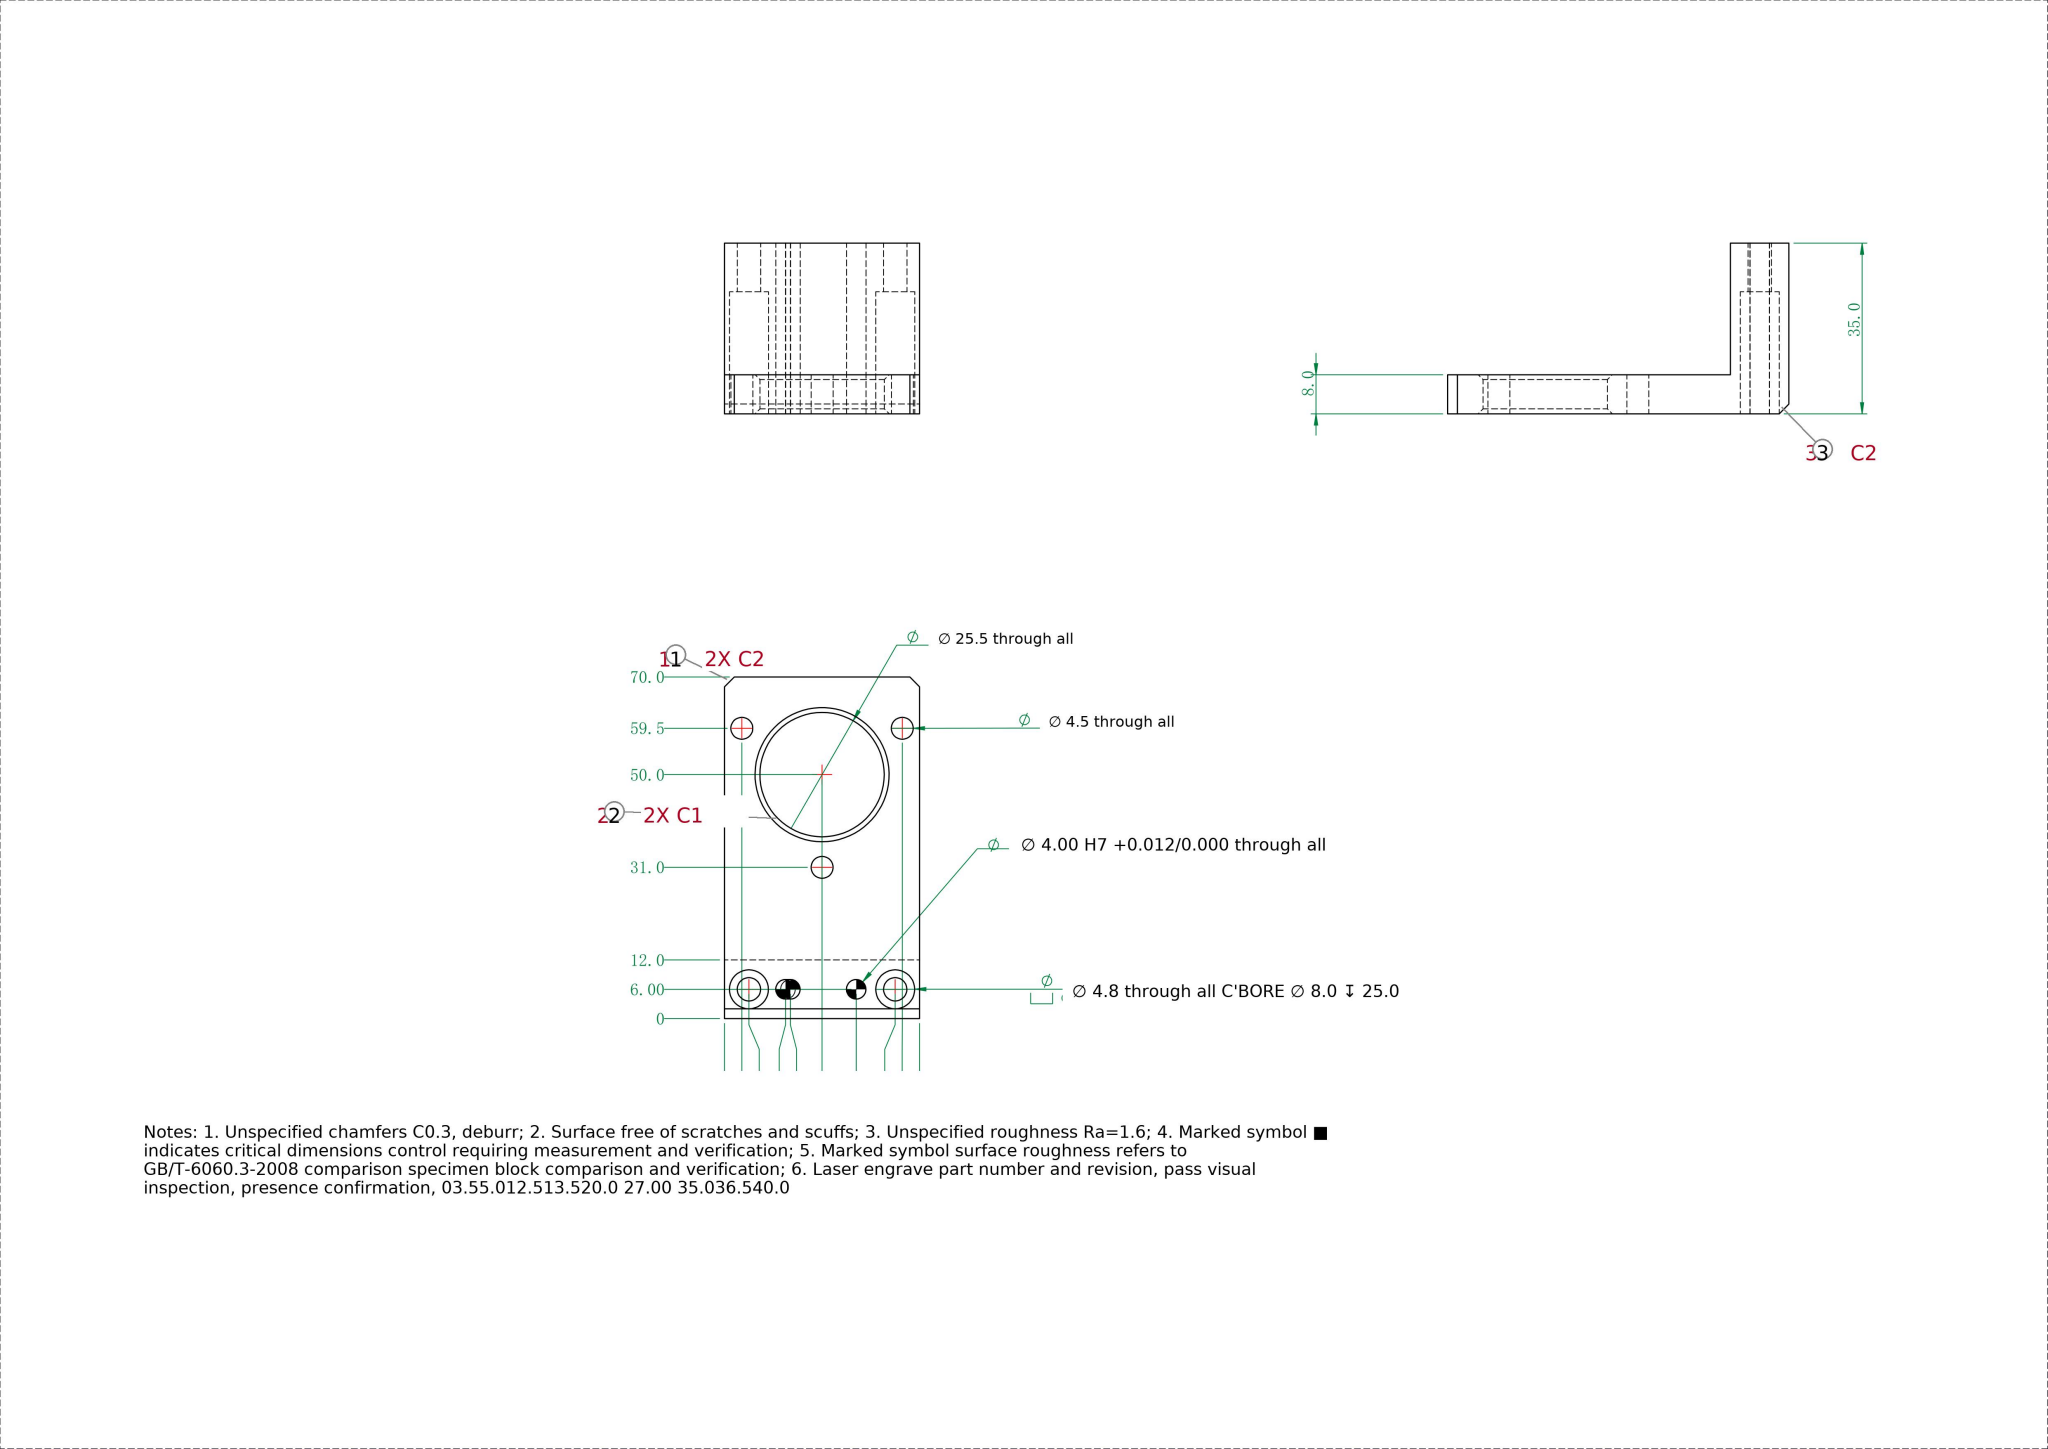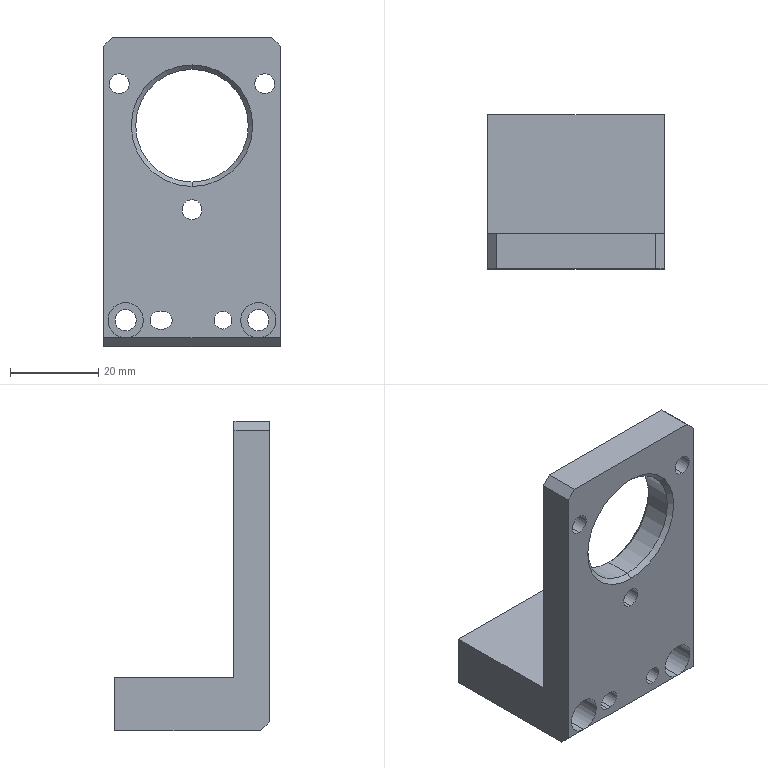Part | SolidWorks | mm | 1 solid | 39 faces | box 40 x 35 x 70 mm | volume 26804 mm3 | cylinder 20 | plane 15 | cone 4 | commonest cylinder face diameters 4.5 x6 4 x4 8 x4 4.8 x4 25.5 x2